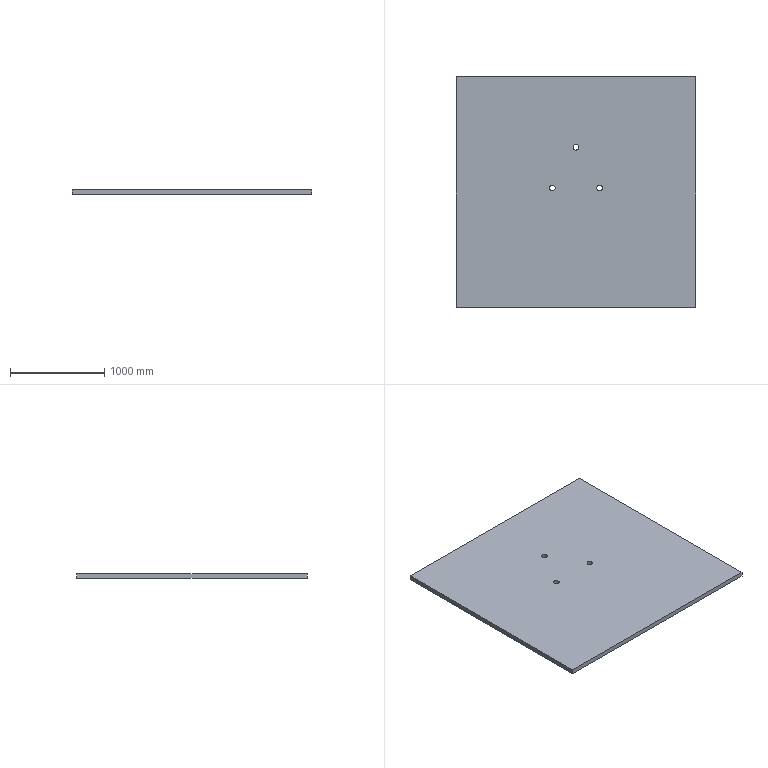Component | NX | Root-owned geometry | 1 solid | 9 faces | box 2530 x 2440 x 50 mm | volume 308235885 mm3 | plane 6 | cylinder 3 | commonest cylinder face diameters 60 x3
STEP:
#1=CARTESIAN_POINT('',(0.,0.,0.));
#2=DIRECTION('',(0.,0.,1.));
#3=DIRECTION('',(1.,0.,0.));
#4=AXIS2_PLACEMENT_3D('',#1,#2,#3);
#5=CARTESIAN_POINT('',(-1170.,950.,-10.));
#6=VERTEX_POINT('',#5);
#7=CARTESIAN_POINT('',(-1170.,-1490.,-10.));
#8=VERTEX_POINT('',#7);
#9=CARTESIAN_POINT('',(-1170.,950.,-10.));
#10=DIRECTION('',(0.,-1.,0.));
#11=VECTOR('',#10,1.);
#12=LINE('',#9,#11);
#13=CARTESIAN_POINT('',(-1170.,950.,-60.));
#14=DIRECTION('',(-1.,0.,0.));
#15=DIRECTION('',(0.,0.,1.));
#16=AXIS2_PLACEMENT_3D('',#13,#14,#15);
#17=PLANE('',#16);
#18=CARTESIAN_POINT('',(50.,0.));
#19=DIRECTION('',(0.,-1.));
#20=VECTOR('',#19,1.);
#21=LINE('',#18,#20);
#22=(GEOMETRIC_REPRESENTATION_CONTEXT(2)PARAMETRIC_REPRESENTATION_CONTEXT()REPRESENTATION_CONTEXT('',''));
#23=DEFINITIONAL_REPRESENTATION('',(#21),#22);
#24=PCURVE('',#17,#23);
#25=CARTESIAN_POINT('',(-156.043,-228.882,-10.));
#26=DIRECTION('',(0.,0.,1.));
#27=DIRECTION('',(1.,0.,0.));
#28=AXIS2_PLACEMENT_3D('',#25,#26,#27);
#29=PLANE('',#28);
#30=CARTESIAN_POINT('',(-1013.957,1178.882));
#31=DIRECTION('',(0.,-1.));
#32=VECTOR('',#31,1.);
#33=LINE('',#30,#32);
#34=(GEOMETRIC_REPRESENTATION_CONTEXT(2)PARAMETRIC_REPRESENTATION_CONTEXT()REPRESENTATION_CONTEXT('',''));
#35=DEFINITIONAL_REPRESENTATION('',(#33),#34);
#36=PCURVE('',#29,#35);
#37=SURFACE_CURVE('',#12,(#24,#36),.PCURVE_S1.);
#38=EDGE_CURVE('',#6,#8,#37,.T.);
#39=ORIENTED_EDGE('',*,*,#38,.F.);
#40=CARTESIAN_POINT('',(-1170.,950.,-60.));
#41=VERTEX_POINT('',#40);
#42=CARTESIAN_POINT('',(-1170.,950.,-60.));
#43=DIRECTION('',(0.,0.,1.));
#44=VECTOR('',#43,1.);
#45=LINE('',#42,#44);
#46=CARTESIAN_POINT('',(0.,0.));
#47=DIRECTION('',(1.,0.));
#48=VECTOR('',#47,1.);
#49=LINE('',#46,#48);
#50=(GEOMETRIC_REPRESENTATION_CONTEXT(2)PARAMETRIC_REPRESENTATION_CONTEXT()REPRESENTATION_CONTEXT('',''));
#51=DEFINITIONAL_REPRESENTATION('',(#49),#50);
#52=PCURVE('',#17,#51);
#53=CARTESIAN_POINT('',(1360.,950.,-60.));
#54=DIRECTION('',(0.,1.,0.));
#55=DIRECTION('',(0.,0.,1.));
#56=AXIS2_PLACEMENT_3D('',#53,#54,#55);
#57=PLANE('',#56);
#58=CARTESIAN_POINT('',(0.,-2530.));
#59=DIRECTION('',(1.,0.));
#60=VECTOR('',#59,1.);
#61=LINE('',#58,#60);
#62=(GEOMETRIC_REPRESENTATION_CONTEXT(2)PARAMETRIC_REPRESENTATION_CONTEXT()REPRESENTATION_CONTEXT('',''));
#63=DEFINITIONAL_REPRESENTATION('',(#61),#62);
#64=PCURVE('',#57,#63);
#65=SURFACE_CURVE('',#45,(#52,#64),.PCURVE_S1.);
#66=EDGE_CURVE('',#41,#6,#65,.T.);
#67=ORIENTED_EDGE('',*,*,#66,.F.);
#68=CARTESIAN_POINT('',(-1170.,-1490.,-60.));
#69=VERTEX_POINT('',#68);
#70=CARTESIAN_POINT('',(-1170.,950.,-60.));
#71=DIRECTION('',(0.,-1.,0.));
#72=VECTOR('',#71,1.);
#73=LINE('',#70,#72);
#74=CARTESIAN_POINT('',(0.,0.));
#75=DIRECTION('',(0.,-1.));
#76=VECTOR('',#75,1.);
#77=LINE('',#74,#76);
#78=(GEOMETRIC_REPRESENTATION_CONTEXT(2)PARAMETRIC_REPRESENTATION_CONTEXT()REPRESENTATION_CONTEXT('',''));
#79=DEFINITIONAL_REPRESENTATION('',(#77),#78);
#80=PCURVE('',#17,#79);
#81=CARTESIAN_POINT('',(-156.043,-228.882,-60.));
#82=DIRECTION('',(0.,0.,1.));
#83=DIRECTION('',(1.,0.,0.));
#84=AXIS2_PLACEMENT_3D('',#81,#82,#83);
#85=PLANE('',#84);
#86=CARTESIAN_POINT('',(-1013.957,1178.882));
#87=DIRECTION('',(0.,-1.));
#88=VECTOR('',#87,1.);
#89=LINE('',#86,#88);
#90=(GEOMETRIC_REPRESENTATION_CONTEXT(2)PARAMETRIC_REPRESENTATION_CONTEXT()REPRESENTATION_CONTEXT('',''));
#91=DEFINITIONAL_REPRESENTATION('',(#89),#90);
#92=PCURVE('',#85,#91);
#93=SURFACE_CURVE('',#73,(#80,#92),.PCURVE_S1.);
#94=EDGE_CURVE('',#41,#69,#93,.T.);
#95=ORIENTED_EDGE('',*,*,#94,.T.);
#96=CARTESIAN_POINT('',(-1170.,-1490.,-60.));
#97=DIRECTION('',(0.,0.,1.));
#98=VECTOR('',#97,1.);
#99=LINE('',#96,#98);
#100=CARTESIAN_POINT('',(0.,-2440.));
#101=DIRECTION('',(1.,0.));
#102=VECTOR('',#101,1.);
#103=LINE('',#100,#102);
#104=(GEOMETRIC_REPRESENTATION_CONTEXT(2)PARAMETRIC_REPRESENTATION_CONTEXT()REPRESENTATION_CONTEXT('',''));
#105=DEFINITIONAL_REPRESENTATION('',(#103),#104);
#106=PCURVE('',#17,#105);
#107=CARTESIAN_POINT('',(-1170.,-1490.,-60.));
#108=DIRECTION('',(0.,-1.,0.));
#109=DIRECTION('',(0.,0.,-1.));
#110=AXIS2_PLACEMENT_3D('',#107,#108,#109);
#111=PLANE('',#110);
#112=CARTESIAN_POINT('',(0.,0.));
#113=DIRECTION('',(-1.,0.));
#114=VECTOR('',#113,1.);
#115=LINE('',#112,#114);
#116=(GEOMETRIC_REPRESENTATION_CONTEXT(2)PARAMETRIC_REPRESENTATION_CONTEXT()REPRESENTATION_CONTEXT('',''));
#117=DEFINITIONAL_REPRESENTATION('',(#115),#116);
#118=PCURVE('',#111,#117);
#119=SURFACE_CURVE('',#99,(#106,#118),.PCURVE_S1.);
#120=EDGE_CURVE('',#69,#8,#119,.T.);
#121=ORIENTED_EDGE('',*,*,#120,.T.);
#122=EDGE_LOOP('',(#39,#67,#95,#121));
#123=FACE_BOUND('',#122,.T.);
#124=ADVANCED_FACE('',(#123),#17,.T.);
#125=CARTESIAN_POINT('',(1360.,-1490.,-10.));
#126=VERTEX_POINT('',#125);
#127=CARTESIAN_POINT('',(-1170.,-1490.,-10.));
#128=DIRECTION('',(1.,0.,0.));
#129=VECTOR('',#128,1.);
#130=LINE('',#127,#129);
#131=CARTESIAN_POINT('',(-50.,0.));
#132=DIRECTION('',(0.,1.));
#133=VECTOR('',#132,1.);
#134=LINE('',#131,#133);
#135=(GEOMETRIC_REPRESENTATION_CONTEXT(2)PARAMETRIC_REPRESENTATION_CONTEXT()REPRESENTATION_CONTEXT('',''));
#136=DEFINITIONAL_REPRESENTATION('',(#134),#135);
#137=PCURVE('',#111,#136);
#138=CARTESIAN_POINT('',(-1013.957,-1261.118));
#139=DIRECTION('',(1.,0.));
#140=VECTOR('',#139,1.);
#141=LINE('',#138,#140);
#142=(GEOMETRIC_REPRESENTATION_CONTEXT(2)PARAMETRIC_REPRESENTATION_CONTEXT()REPRESENTATION_CONTEXT('',''));
#143=DEFINITIONAL_REPRESENTATION('',(#141),#142);
#144=PCURVE('',#29,#143);
#145=SURFACE_CURVE('',#130,(#137,#144),.PCURVE_S1.);
#146=EDGE_CURVE('',#8,#126,#145,.T.);
#147=ORIENTED_EDGE('',*,*,#146,.F.);
#148=ORIENTED_EDGE('',*,*,#120,.F.);
#149=CARTESIAN_POINT('',(1360.,-1490.,-60.));
#150=VERTEX_POINT('',#149);
#151=CARTESIAN_POINT('',(-1170.,-1490.,-60.));
#152=DIRECTION('',(1.,0.,0.));
#153=VECTOR('',#152,1.);
#154=LINE('',#151,#153);
#155=CARTESIAN_POINT('',(0.,0.));
#156=DIRECTION('',(0.,1.));
#157=VECTOR('',#156,1.);
#158=LINE('',#155,#157);
#159=(GEOMETRIC_REPRESENTATION_CONTEXT(2)PARAMETRIC_REPRESENTATION_CONTEXT()REPRESENTATION_CONTEXT('',''));
#160=DEFINITIONAL_REPRESENTATION('',(#158),#159);
#161=PCURVE('',#111,#160);
#162=CARTESIAN_POINT('',(-1013.957,-1261.118));
#163=DIRECTION('',(1.,0.));
#164=VECTOR('',#163,1.);
#165=LINE('',#162,#164);
#166=(GEOMETRIC_REPRESENTATION_CONTEXT(2)PARAMETRIC_REPRESENTATION_CONTEXT()REPRESENTATION_CONTEXT('',''));
#167=DEFINITIONAL_REPRESENTATION('',(#165),#166);
#168=PCURVE('',#85,#167);
#169=SURFACE_CURVE('',#154,(#161,#168),.PCURVE_S1.);
#170=EDGE_CURVE('',#69,#150,#169,.T.);
#171=ORIENTED_EDGE('',*,*,#170,.T.);
#172=CARTESIAN_POINT('',(1360.,-1490.,-60.));
#173=DIRECTION('',(0.,0.,1.));
#174=VECTOR('',#173,1.);
#175=LINE('',#172,#174);
#176=CARTESIAN_POINT('',(0.,2530.));
#177=DIRECTION('',(-1.,0.));
#178=VECTOR('',#177,1.);
#179=LINE('',#176,#178);
#180=(GEOMETRIC_REPRESENTATION_CONTEXT(2)PARAMETRIC_REPRESENTATION_CONTEXT()REPRESENTATION_CONTEXT('',''));
#181=DEFINITIONAL_REPRESENTATION('',(#179),#180);
#182=PCURVE('',#111,#181);
#183=CARTESIAN_POINT('',(1360.,-1490.,-60.));
#184=DIRECTION('',(1.,0.,0.));
#185=DIRECTION('',(0.,0.,-1.));
#186=AXIS2_PLACEMENT_3D('',#183,#184,#185);
#187=PLANE('',#186);
#188=CARTESIAN_POINT('',(0.,0.));
#189=DIRECTION('',(-1.,0.));
#190=VECTOR('',#189,1.);
#191=LINE('',#188,#190);
#192=(GEOMETRIC_REPRESENTATION_CONTEXT(2)PARAMETRIC_REPRESENTATION_CONTEXT()REPRESENTATION_CONTEXT('',''));
#193=DEFINITIONAL_REPRESENTATION('',(#191),#192);
#194=PCURVE('',#187,#193);
#195=SURFACE_CURVE('',#175,(#182,#194),.PCURVE_S1.);
#196=EDGE_CURVE('',#150,#126,#195,.T.);
#197=ORIENTED_EDGE('',*,*,#196,.T.);
#198=EDGE_LOOP('',(#147,#148,#171,#197));
#199=FACE_BOUND('',#198,.T.);
#200=ADVANCED_FACE('',(#199),#111,.T.);
#201=CARTESIAN_POINT('',(1360.,950.,-10.));
#202=VERTEX_POINT('',#201);
#203=CARTESIAN_POINT('',(1360.,-1490.,-10.));
#204=DIRECTION('',(0.,1.,0.));
#205=VECTOR('',#204,1.);
#206=LINE('',#203,#205);
#207=CARTESIAN_POINT('',(-50.,0.));
#208=DIRECTION('',(0.,1.));
#209=VECTOR('',#208,1.);
#210=LINE('',#207,#209);
#211=(GEOMETRIC_REPRESENTATION_CONTEXT(2)PARAMETRIC_REPRESENTATION_CONTEXT()REPRESENTATION_CONTEXT('',''));
#212=DEFINITIONAL_REPRESENTATION('',(#210),#211);
#213=PCURVE('',#187,#212);
#214=CARTESIAN_POINT('',(1516.043,-1261.118));
#215=DIRECTION('',(0.,1.));
#216=VECTOR('',#215,1.);
#217=LINE('',#214,#216);
#218=(GEOMETRIC_REPRESENTATION_CONTEXT(2)PARAMETRIC_REPRESENTATION_CONTEXT()REPRESENTATION_CONTEXT('',''));
#219=DEFINITIONAL_REPRESENTATION('',(#217),#218);
#220=PCURVE('',#29,#219);
#221=SURFACE_CURVE('',#206,(#213,#220),.PCURVE_S1.);
#222=EDGE_CURVE('',#126,#202,#221,.T.);
#223=ORIENTED_EDGE('',*,*,#222,.F.);
#224=ORIENTED_EDGE('',*,*,#196,.F.);
#225=CARTESIAN_POINT('',(1360.,950.,-60.));
#226=VERTEX_POINT('',#225);
#227=CARTESIAN_POINT('',(1360.,-1490.,-60.));
#228=DIRECTION('',(0.,1.,0.));
#229=VECTOR('',#228,1.);
#230=LINE('',#227,#229);
#231=CARTESIAN_POINT('',(0.,0.));
#232=DIRECTION('',(0.,1.));
#233=VECTOR('',#232,1.);
#234=LINE('',#231,#233);
#235=(GEOMETRIC_REPRESENTATION_CONTEXT(2)PARAMETRIC_REPRESENTATION_CONTEXT()REPRESENTATION_CONTEXT('',''));
#236=DEFINITIONAL_REPRESENTATION('',(#234),#235);
#237=PCURVE('',#187,#236);
#238=CARTESIAN_POINT('',(1516.043,-1261.118));
#239=DIRECTION('',(0.,1.));
#240=VECTOR('',#239,1.);
#241=LINE('',#238,#240);
#242=(GEOMETRIC_REPRESENTATION_CONTEXT(2)PARAMETRIC_REPRESENTATION_CONTEXT()REPRESENTATION_CONTEXT('',''));
#243=DEFINITIONAL_REPRESENTATION('',(#241),#242);
#244=PCURVE('',#85,#243);
#245=SURFACE_CURVE('',#230,(#237,#244),.PCURVE_S1.);
#246=EDGE_CURVE('',#150,#226,#245,.T.);
#247=ORIENTED_EDGE('',*,*,#246,.T.);
#248=CARTESIAN_POINT('',(1360.,950.,-60.));
#249=DIRECTION('',(0.,0.,1.));
#250=VECTOR('',#249,1.);
#251=LINE('',#248,#250);
#252=CARTESIAN_POINT('',(0.,2440.));
#253=DIRECTION('',(-1.,0.));
#254=VECTOR('',#253,1.);
#255=LINE('',#252,#254);
#256=(GEOMETRIC_REPRESENTATION_CONTEXT(2)PARAMETRIC_REPRESENTATION_CONTEXT()REPRESENTATION_CONTEXT('',''));
#257=DEFINITIONAL_REPRESENTATION('',(#255),#256);
#258=PCURVE('',#187,#257);
#259=CARTESIAN_POINT('',(0.,0.));
#260=DIRECTION('',(1.,0.));
#261=VECTOR('',#260,1.);
#262=LINE('',#259,#261);
#263=(GEOMETRIC_REPRESENTATION_CONTEXT(2)PARAMETRIC_REPRESENTATION_CONTEXT()REPRESENTATION_CONTEXT('',''));
#264=DEFINITIONAL_REPRESENTATION('',(#262),#263);
#265=PCURVE('',#57,#264);
#266=SURFACE_CURVE('',#251,(#258,#265),.PCURVE_S1.);
#267=EDGE_CURVE('',#226,#202,#266,.T.);
#268=ORIENTED_EDGE('',*,*,#267,.T.);
#269=EDGE_LOOP('',(#223,#224,#247,#268));
#270=FACE_BOUND('',#269,.T.);
#271=ADVANCED_FACE('',(#270),#187,.T.);
#272=CARTESIAN_POINT('',(123.957,203.937,-60.));
#273=VERTEX_POINT('',#272);
#274=CARTESIAN_POINT('',(93.957,203.937,-60.));
#275=DIRECTION('',(0.,0.,1.));
#276=DIRECTION('',(1.,0.,0.));
#277=AXIS2_PLACEMENT_3D('',#274,#275,#276);
#278=CIRCLE('',#277,30.);
#279=CARTESIAN_POINT('',(93.957,203.937,-60.));
#280=DIRECTION('',(0.,0.,1.));
#281=DIRECTION('',(1.,0.,0.));
#282=AXIS2_PLACEMENT_3D('',#279,#280,#281);
#283=CYLINDRICAL_SURFACE('',#282,30.);
#284=CARTESIAN_POINT('',(0.,0.));
#285=DIRECTION('',(1.,0.));
#286=VECTOR('',#285,1.);
#287=LINE('',#284,#286);
#288=(GEOMETRIC_REPRESENTATION_CONTEXT(2)PARAMETRIC_REPRESENTATION_CONTEXT()REPRESENTATION_CONTEXT('',''));
#289=DEFINITIONAL_REPRESENTATION('',(#287),#288);
#290=PCURVE('',#283,#289);
#291=CARTESIAN_POINT('',(250.,432.819));
#292=DIRECTION('',(1.,0.));
#293=AXIS2_PLACEMENT_2D('',#291,#292);
#294=CIRCLE('',#293,30.);
#295=(GEOMETRIC_REPRESENTATION_CONTEXT(2)PARAMETRIC_REPRESENTATION_CONTEXT()REPRESENTATION_CONTEXT('',''));
#296=DEFINITIONAL_REPRESENTATION('',(#294),#295);
#297=PCURVE('',#85,#296);
#298=SURFACE_CURVE('',#278,(#290,#297),.PCURVE_S1.);
#299=EDGE_CURVE('',#273,#273,#298,.T.);
#300=ORIENTED_EDGE('',*,*,#299,.T.);
#301=CARTESIAN_POINT('',(123.957,203.937,-10.));
#302=VERTEX_POINT('',#301);
#303=CARTESIAN_POINT('',(123.957,203.937,-60.));
#304=CARTESIAN_POINT('',(123.957,203.937,-10.));
#305=B_SPLINE_CURVE_WITH_KNOTS('',1,(#303,#304),.UNSPECIFIED.,.F.,.F.,(2,2),(0.,50.),.PIECEWISE_BEZIER_KNOTS.);
#306=CARTESIAN_POINT('',(6.283,0.));
#307=DIRECTION('',(0.,1.));
#308=VECTOR('',#307,1.);
#309=LINE('',#306,#308);
#310=(GEOMETRIC_REPRESENTATION_CONTEXT(2)PARAMETRIC_REPRESENTATION_CONTEXT()REPRESENTATION_CONTEXT('',''));
#311=DEFINITIONAL_REPRESENTATION('',(#309),#310);
#312=PCURVE('',#283,#311);
#313=CARTESIAN_POINT('',(0.,0.));
#314=DIRECTION('',(0.,1.));
#315=VECTOR('',#314,1.);
#316=LINE('',#313,#315);
#317=(GEOMETRIC_REPRESENTATION_CONTEXT(2)PARAMETRIC_REPRESENTATION_CONTEXT()REPRESENTATION_CONTEXT('',''));
#318=DEFINITIONAL_REPRESENTATION('',(#316),#317);
#319=PCURVE('',#283,#318);
#320=SEAM_CURVE('',#305,(#312,#319),.PCURVE_S1.);
#321=EDGE_CURVE('',#273,#302,#320,.T.);
#322=ORIENTED_EDGE('',*,*,#321,.T.);
#323=CARTESIAN_POINT('',(93.957,203.937,-10.));
#324=DIRECTION('',(0.,0.,1.));
#325=DIRECTION('',(1.,0.,0.));
#326=AXIS2_PLACEMENT_3D('',#323,#324,#325);
#327=CIRCLE('',#326,30.);
#328=CARTESIAN_POINT('',(0.,50.));
#329=DIRECTION('',(1.,0.));
#330=VECTOR('',#329,1.);
#331=LINE('',#328,#330);
#332=(GEOMETRIC_REPRESENTATION_CONTEXT(2)PARAMETRIC_REPRESENTATION_CONTEXT()REPRESENTATION_CONTEXT('',''));
#333=DEFINITIONAL_REPRESENTATION('',(#331),#332);
#334=PCURVE('',#283,#333);
#335=CARTESIAN_POINT('',(250.,432.819));
#336=DIRECTION('',(1.,0.));
#337=AXIS2_PLACEMENT_2D('',#335,#336);
#338=CIRCLE('',#337,30.);
#339=(GEOMETRIC_REPRESENTATION_CONTEXT(2)PARAMETRIC_REPRESENTATION_CONTEXT()REPRESENTATION_CONTEXT('',''));
#340=DEFINITIONAL_REPRESENTATION('',(#338),#339);
#341=PCURVE('',#29,#340);
#342=SURFACE_CURVE('',#327,(#334,#341),.PCURVE_S1.);
#343=EDGE_CURVE('',#302,#302,#342,.T.);
#344=ORIENTED_EDGE('',*,*,#343,.F.);
#345=ORIENTED_EDGE('',*,*,#321,.F.);
#346=EDGE_LOOP('',(#300,#322,#344,#345));
#347=FACE_BOUND('',#346,.F.);
#348=ADVANCED_FACE('',(#347),#283,.F.);
#349=CARTESIAN_POINT('',(-126.043,-228.882,-60.));
#350=VERTEX_POINT('',#349);
#351=CARTESIAN_POINT('',(-156.043,-228.882,-60.));
#352=DIRECTION('',(0.,0.,1.));
#353=DIRECTION('',(1.,0.,0.));
#354=AXIS2_PLACEMENT_3D('',#351,#352,#353);
#355=CIRCLE('',#354,30.);
#356=CARTESIAN_POINT('',(-156.043,-228.882,-60.));
#357=DIRECTION('',(0.,0.,1.));
#358=DIRECTION('',(1.,0.,0.));
#359=AXIS2_PLACEMENT_3D('',#356,#357,#358);
#360=CYLINDRICAL_SURFACE('',#359,30.);
#361=CARTESIAN_POINT('',(0.,0.));
#362=DIRECTION('',(1.,0.));
#363=VECTOR('',#362,1.);
#364=LINE('',#361,#363);
#365=(GEOMETRIC_REPRESENTATION_CONTEXT(2)PARAMETRIC_REPRESENTATION_CONTEXT()REPRESENTATION_CONTEXT('',''));
#366=DEFINITIONAL_REPRESENTATION('',(#364),#365);
#367=PCURVE('',#360,#366);
#368=CARTESIAN_POINT('',(0.,0.));
#369=DIRECTION('',(1.,0.));
#370=AXIS2_PLACEMENT_2D('',#368,#369);
#371=CIRCLE('',#370,30.);
#372=(GEOMETRIC_REPRESENTATION_CONTEXT(2)PARAMETRIC_REPRESENTATION_CONTEXT()REPRESENTATION_CONTEXT('',''));
#373=DEFINITIONAL_REPRESENTATION('',(#371),#372);
#374=PCURVE('',#85,#373);
#375=SURFACE_CURVE('',#355,(#367,#374),.PCURVE_S1.);
#376=EDGE_CURVE('',#350,#350,#375,.T.);
#377=ORIENTED_EDGE('',*,*,#376,.T.);
#378=CARTESIAN_POINT('',(-126.043,-228.882,-10.));
#379=VERTEX_POINT('',#378);
#380=CARTESIAN_POINT('',(-126.043,-228.882,-60.));
#381=CARTESIAN_POINT('',(-126.043,-228.882,-10.));
#382=B_SPLINE_CURVE_WITH_KNOTS('',1,(#380,#381),.UNSPECIFIED.,.F.,.F.,(2,2),(0.,50.),.PIECEWISE_BEZIER_KNOTS.);
#383=CARTESIAN_POINT('',(6.283,0.));
#384=DIRECTION('',(0.,1.));
#385=VECTOR('',#384,1.);
#386=LINE('',#383,#385);
#387=(GEOMETRIC_REPRESENTATION_CONTEXT(2)PARAMETRIC_REPRESENTATION_CONTEXT()REPRESENTATION_CONTEXT('',''));
#388=DEFINITIONAL_REPRESENTATION('',(#386),#387);
#389=PCURVE('',#360,#388);
#390=CARTESIAN_POINT('',(0.,0.));
#391=DIRECTION('',(0.,1.));
#392=VECTOR('',#391,1.);
#393=LINE('',#390,#392);
#394=(GEOMETRIC_REPRESENTATION_CONTEXT(2)PARAMETRIC_REPRESENTATION_CONTEXT()REPRESENTATION_CONTEXT('',''));
#395=DEFINITIONAL_REPRESENTATION('',(#393),#394);
#396=PCURVE('',#360,#395);
#397=SEAM_CURVE('',#382,(#389,#396),.PCURVE_S1.);
#398=EDGE_CURVE('',#350,#379,#397,.T.);
#399=ORIENTED_EDGE('',*,*,#398,.T.);
#400=CARTESIAN_POINT('',(-156.043,-228.882,-10.));
#401=DIRECTION('',(0.,0.,1.));
#402=DIRECTION('',(1.,0.,0.));
#403=AXIS2_PLACEMENT_3D('',#400,#401,#402);
#404=CIRCLE('',#403,30.);
#405=CARTESIAN_POINT('',(0.,50.));
#406=DIRECTION('',(1.,0.));
#407=VECTOR('',#406,1.);
#408=LINE('',#405,#407);
#409=(GEOMETRIC_REPRESENTATION_CONTEXT(2)PARAMETRIC_REPRESENTATION_CONTEXT()REPRESENTATION_CONTEXT('',''));
#410=DEFINITIONAL_REPRESENTATION('',(#408),#409);
#411=PCURVE('',#360,#410);
#412=CARTESIAN_POINT('',(0.,0.));
#413=DIRECTION('',(1.,0.));
#414=AXIS2_PLACEMENT_2D('',#412,#413);
#415=CIRCLE('',#414,30.);
#416=(GEOMETRIC_REPRESENTATION_CONTEXT(2)PARAMETRIC_REPRESENTATION_CONTEXT()REPRESENTATION_CONTEXT('',''));
#417=DEFINITIONAL_REPRESENTATION('',(#415),#416);
#418=PCURVE('',#29,#417);
#419=SURFACE_CURVE('',#404,(#411,#418),.PCURVE_S1.);
#420=EDGE_CURVE('',#379,#379,#419,.T.);
#421=ORIENTED_EDGE('',*,*,#420,.F.);
#422=ORIENTED_EDGE('',*,*,#398,.F.);
#423=EDGE_LOOP('',(#377,#399,#421,#422));
#424=FACE_BOUND('',#423,.F.);
#425=ADVANCED_FACE('',(#424),#360,.F.);
#426=CARTESIAN_POINT('',(1360.,950.,-10.));
#427=DIRECTION('',(-1.,0.,0.));
#428=VECTOR('',#427,1.);
#429=LINE('',#426,#428);
#430=CARTESIAN_POINT('',(50.,0.));
#431=DIRECTION('',(0.,-1.));
#432=VECTOR('',#431,1.);
#433=LINE('',#430,#432);
#434=(GEOMETRIC_REPRESENTATION_CONTEXT(2)PARAMETRIC_REPRESENTATION_CONTEXT()REPRESENTATION_CONTEXT('',''));
#435=DEFINITIONAL_REPRESENTATION('',(#433),#434);
#436=PCURVE('',#57,#435);
#437=CARTESIAN_POINT('',(1516.043,1178.882));
#438=DIRECTION('',(-1.,0.));
#439=VECTOR('',#438,1.);
#440=LINE('',#437,#439);
#441=(GEOMETRIC_REPRESENTATION_CONTEXT(2)PARAMETRIC_REPRESENTATION_CONTEXT()REPRESENTATION_CONTEXT('',''));
#442=DEFINITIONAL_REPRESENTATION('',(#440),#441);
#443=PCURVE('',#29,#442);
#444=SURFACE_CURVE('',#429,(#436,#443),.PCURVE_S1.);
#445=EDGE_CURVE('',#202,#6,#444,.T.);
#446=ORIENTED_EDGE('',*,*,#445,.F.);
#447=ORIENTED_EDGE('',*,*,#267,.F.);
#448=CARTESIAN_POINT('',(1360.,950.,-60.));
#449=DIRECTION('',(-1.,0.,0.));
#450=VECTOR('',#449,1.);
#451=LINE('',#448,#450);
#452=CARTESIAN_POINT('',(0.,0.));
#453=DIRECTION('',(0.,-1.));
#454=VECTOR('',#453,1.);
#455=LINE('',#452,#454);
#456=(GEOMETRIC_REPRESENTATION_CONTEXT(2)PARAMETRIC_REPRESENTATION_CONTEXT()REPRESENTATION_CONTEXT('',''));
#457=DEFINITIONAL_REPRESENTATION('',(#455),#456);
#458=PCURVE('',#57,#457);
#459=CARTESIAN_POINT('',(1516.043,1178.882));
#460=DIRECTION('',(-1.,0.));
#461=VECTOR('',#460,1.);
#462=LINE('',#459,#461);
#463=(GEOMETRIC_REPRESENTATION_CONTEXT(2)PARAMETRIC_REPRESENTATION_CONTEXT()REPRESENTATION_CONTEXT('',''));
#464=DEFINITIONAL_REPRESENTATION('',(#462),#463);
#465=PCURVE('',#85,#464);
#466=SURFACE_CURVE('',#451,(#458,#465),.PCURVE_S1.);
#467=EDGE_CURVE('',#226,#41,#466,.T.);
#468=ORIENTED_EDGE('',*,*,#467,.T.);
#469=ORIENTED_EDGE('',*,*,#66,.T.);
#470=EDGE_LOOP('',(#446,#447,#468,#469));
#471=FACE_BOUND('',#470,.T.);
#472=ADVANCED_FACE('',(#471),#57,.T.);
#473=CARTESIAN_POINT('',(373.957,-228.882,-60.));
#474=VERTEX_POINT('',#473);
#475=CARTESIAN_POINT('',(343.957,-228.882,-60.));
#476=DIRECTION('',(0.,0.,1.));
#477=DIRECTION('',(1.,0.,0.));
#478=AXIS2_PLACEMENT_3D('',#475,#476,#477);
#479=CIRCLE('',#478,30.);
#480=CARTESIAN_POINT('',(343.957,-228.882,-60.));
#481=DIRECTION('',(0.,0.,1.));
#482=DIRECTION('',(1.,0.,0.));
#483=AXIS2_PLACEMENT_3D('',#480,#481,#482);
#484=CYLINDRICAL_SURFACE('',#483,30.);
#485=CARTESIAN_POINT('',(0.,0.));
#486=DIRECTION('',(1.,0.));
#487=VECTOR('',#486,1.);
#488=LINE('',#485,#487);
#489=(GEOMETRIC_REPRESENTATION_CONTEXT(2)PARAMETRIC_REPRESENTATION_CONTEXT()REPRESENTATION_CONTEXT('',''));
#490=DEFINITIONAL_REPRESENTATION('',(#488),#489);
#491=PCURVE('',#484,#490);
#492=CARTESIAN_POINT('',(500.,-0.));
#493=DIRECTION('',(1.,0.));
#494=AXIS2_PLACEMENT_2D('',#492,#493);
#495=CIRCLE('',#494,30.);
#496=(GEOMETRIC_REPRESENTATION_CONTEXT(2)PARAMETRIC_REPRESENTATION_CONTEXT()REPRESENTATION_CONTEXT('',''));
#497=DEFINITIONAL_REPRESENTATION('',(#495),#496);
#498=PCURVE('',#85,#497);
#499=SURFACE_CURVE('',#479,(#491,#498),.PCURVE_S1.);
#500=EDGE_CURVE('',#474,#474,#499,.T.);
#501=ORIENTED_EDGE('',*,*,#500,.T.);
#502=CARTESIAN_POINT('',(373.957,-228.882,-10.));
#503=VERTEX_POINT('',#502);
#504=CARTESIAN_POINT('',(373.957,-228.882,-60.));
#505=CARTESIAN_POINT('',(373.957,-228.882,-10.));
#506=B_SPLINE_CURVE_WITH_KNOTS('',1,(#504,#505),.UNSPECIFIED.,.F.,.F.,(2,2),(0.,50.),.PIECEWISE_BEZIER_KNOTS.);
#507=CARTESIAN_POINT('',(6.283,0.));
#508=DIRECTION('',(0.,1.));
#509=VECTOR('',#508,1.);
#510=LINE('',#507,#509);
#511=(GEOMETRIC_REPRESENTATION_CONTEXT(2)PARAMETRIC_REPRESENTATION_CONTEXT()REPRESENTATION_CONTEXT('',''));
#512=DEFINITIONAL_REPRESENTATION('',(#510),#511);
#513=PCURVE('',#484,#512);
#514=CARTESIAN_POINT('',(0.,0.));
#515=DIRECTION('',(0.,1.));
#516=VECTOR('',#515,1.);
#517=LINE('',#514,#516);
#518=(GEOMETRIC_REPRESENTATION_CONTEXT(2)PARAMETRIC_REPRESENTATION_CONTEXT()REPRESENTATION_CONTEXT('',''));
#519=DEFINITIONAL_REPRESENTATION('',(#517),#518);
#520=PCURVE('',#484,#519);
#521=SEAM_CURVE('',#506,(#513,#520),.PCURVE_S1.);
#522=EDGE_CURVE('',#474,#503,#521,.T.);
#523=ORIENTED_EDGE('',*,*,#522,.T.);
#524=CARTESIAN_POINT('',(343.957,-228.882,-10.));
#525=DIRECTION('',(0.,0.,1.));
#526=DIRECTION('',(1.,0.,0.));
#527=AXIS2_PLACEMENT_3D('',#524,#525,#526);
#528=CIRCLE('',#527,30.);
#529=CARTESIAN_POINT('',(0.,50.));
#530=DIRECTION('',(1.,0.));
#531=VECTOR('',#530,1.);
#532=LINE('',#529,#531);
#533=(GEOMETRIC_REPRESENTATION_CONTEXT(2)PARAMETRIC_REPRESENTATION_CONTEXT()REPRESENTATION_CONTEXT('',''));
#534=DEFINITIONAL_REPRESENTATION('',(#532),#533);
#535=PCURVE('',#484,#534);
#536=CARTESIAN_POINT('',(500.,-0.));
#537=DIRECTION('',(1.,0.));
#538=AXIS2_PLACEMENT_2D('',#536,#537);
#539=CIRCLE('',#538,30.);
#540=(GEOMETRIC_REPRESENTATION_CONTEXT(2)PARAMETRIC_REPRESENTATION_CONTEXT()REPRESENTATION_CONTEXT('',''));
#541=DEFINITIONAL_REPRESENTATION('',(#539),#540);
#542=PCURVE('',#29,#541);
#543=SURFACE_CURVE('',#528,(#535,#542),.PCURVE_S1.);
#544=EDGE_CURVE('',#503,#503,#543,.T.);
#545=ORIENTED_EDGE('',*,*,#544,.F.);
#546=ORIENTED_EDGE('',*,*,#522,.F.);
#547=EDGE_LOOP('',(#501,#523,#545,#546));
#548=FACE_BOUND('',#547,.F.);
#549=ADVANCED_FACE('',(#548),#484,.F.);
#550=ORIENTED_EDGE('',*,*,#94,.F.);
#551=ORIENTED_EDGE('',*,*,#467,.F.);
#552=ORIENTED_EDGE('',*,*,#246,.F.);
#553=ORIENTED_EDGE('',*,*,#170,.F.);
#554=EDGE_LOOP('',(#550,#551,#552,#553));
#555=FACE_BOUND('',#554,.T.);
#556=ORIENTED_EDGE('',*,*,#376,.T.);
#557=EDGE_LOOP('',(#556));
#558=FACE_BOUND('',#557,.T.);
#559=ORIENTED_EDGE('',*,*,#299,.T.);
#560=EDGE_LOOP('',(#559));
#561=FACE_BOUND('',#560,.T.);
#562=ORIENTED_EDGE('',*,*,#500,.T.);
#563=EDGE_LOOP('',(#562));
#564=FACE_BOUND('',#563,.T.);
#565=ADVANCED_FACE('',(#555,#558,#561,#564),#85,.F.);
#566=ORIENTED_EDGE('',*,*,#38,.T.);
#567=ORIENTED_EDGE('',*,*,#146,.T.);
#568=ORIENTED_EDGE('',*,*,#222,.T.);
#569=ORIENTED_EDGE('',*,*,#445,.T.);
#570=EDGE_LOOP('',(#566,#567,#568,#569));
#571=FACE_BOUND('',#570,.T.);
#572=ORIENTED_EDGE('',*,*,#420,.F.);
#573=EDGE_LOOP('',(#572));
#574=FACE_BOUND('',#573,.T.);
#575=ORIENTED_EDGE('',*,*,#343,.F.);
#576=EDGE_LOOP('',(#575));
#577=FACE_BOUND('',#576,.T.);
#578=ORIENTED_EDGE('',*,*,#544,.F.);
#579=EDGE_LOOP('',(#578));
#580=FACE_BOUND('',#579,.T.);
#581=ADVANCED_FACE('',(#571,#574,#577,#580),#29,.T.);
#582=CLOSED_SHELL('',(#124,#200,#271,#348,#425,#472,#549,#565,#581));
#583=MANIFOLD_SOLID_BREP('',#582);
#584=(LENGTH_UNIT()NAMED_UNIT(*)SI_UNIT(.MILLI.,.METRE.));
#585=UNCERTAINTY_MEASURE_WITH_UNIT(LENGTH_MEASURE(0.000002),#584,'','');
#586=(NAMED_UNIT(*)PLANE_ANGLE_UNIT()SI_UNIT($,.RADIAN.));
#587=(NAMED_UNIT(*)SI_UNIT($,.STERADIAN.)SOLID_ANGLE_UNIT());
#588=(GEOMETRIC_REPRESENTATION_CONTEXT(3)GLOBAL_UNCERTAINTY_ASSIGNED_CONTEXT((#585))GLOBAL_UNIT_ASSIGNED_CONTEXT((#584,#586,#587))REPRESENTATION_CONTEXT('',''));
#589=ADVANCED_BREP_SHAPE_REPRESENTATION('',(#4,#583),#588);